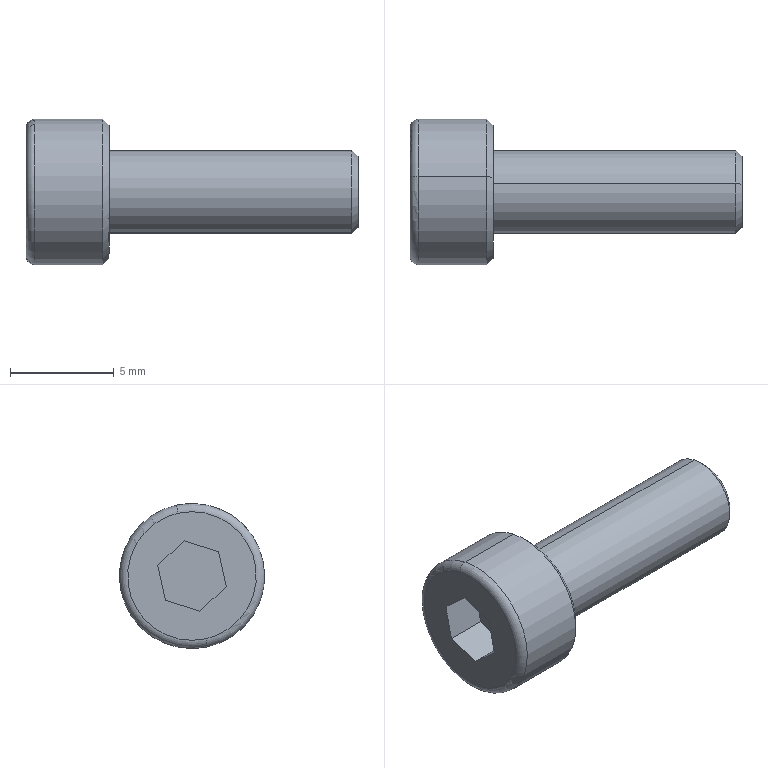Component | SolidWorks | SocketHeadCapScrew_M4_12-1 | 1 solid | 20 faces | box 16 x 7 x 7 mm | volume 287 mm3 | plane 10 | cone 4 | cylinder 4 | torus 2 | commonest cylinder face diameters 7 x2 4 x2
STEP:
#1=COLOUR_RGB('',0.7922,0.8196,0.9333);
#2=FILL_AREA_STYLE_COLOUR('',#1);
#3=FILL_AREA_STYLE('',(#2));
#4=SURFACE_STYLE_FILL_AREA(#3);
#5=SURFACE_SIDE_STYLE('',(#4));
#6=SURFACE_STYLE_USAGE(.BOTH.,#5);
#7=PRESENTATION_STYLE_ASSIGNMENT((#6));
#8=CARTESIAN_POINT('',(-0.1102,-0.2042,-1.204));
#9=VERTEX_POINT('',#8);
#10=CARTESIAN_POINT('',(-0.1102,-0.1502,-0.9575));
#11=VERTEX_POINT('',#10);
#12=CARTESIAN_POINT('',(-0.1102,-0.1772,-1.081));
#13=DIRECTION('',(1.,-0.,-0.));
#14=DIRECTION('',(0.,0.2142,0.9768));
#15=AXIS2_PLACEMENT_3D('',#12,#13,#14);
#16=CIRCLE('',#15,0.126);
#17=EDGE_CURVE('',#9,#11,#16,.T.);
#18=ORIENTED_EDGE('',*,*,#17,.F.);
#19=CARTESIAN_POINT('',(-0.122,-0.2067,-1.215));
#20=VERTEX_POINT('',#19);
#21=CARTESIAN_POINT('',(-0.122,-0.2067,-1.215));
#22=DIRECTION('',(-0.7071,-0.1515,-0.6907));
#23=VECTOR('',#22,39.37);
#24=LINE('',#21,#23);
#25=EDGE_CURVE('',#9,#20,#24,.T.);
#26=ORIENTED_EDGE('',*,*,#25,.T.);
#27=CARTESIAN_POINT('',(-0.122,-0.1476,-0.946));
#28=VERTEX_POINT('',#27);
#29=CARTESIAN_POINT('',(-0.122,-0.1772,-1.081));
#30=DIRECTION('',(-1.,0.,0.));
#31=DIRECTION('',(0.,0.2142,0.9768));
#32=AXIS2_PLACEMENT_3D('',#29,#30,#31);
#33=CIRCLE('',#32,0.1378);
#34=EDGE_CURVE('',#28,#20,#33,.T.);
#35=ORIENTED_EDGE('',*,*,#34,.F.);
#36=CARTESIAN_POINT('',(-0.122,-0.1476,-0.946));
#37=DIRECTION('',(-0.7071,0.1515,0.6907));
#38=VECTOR('',#37,39.37);
#39=LINE('',#36,#38);
#40=EDGE_CURVE('',#11,#28,#39,.T.);
#41=ORIENTED_EDGE('',*,*,#40,.F.);
#42=EDGE_LOOP('',(#18,#26,#35,#41));
#43=FACE_OUTER_BOUND('',#42,.T.);
#44=CARTESIAN_POINT('',(-0.122,-0.1772,-1.081));
#45=DIRECTION('',(-1.,0.,0.));
#46=DIRECTION('',(0.,0.2142,0.9768));
#47=AXIS2_PLACEMENT_3D('',#44,#45,#46);
#48=CONICAL_SURFACE('',#47,0.1378,0.7854);
#49=ADVANCED_FACE('',(#43),#48,.T.);
#50=CARTESIAN_POINT('',(0.3622,-0.1915,-1.146));
#51=VERTEX_POINT('',#50);
#52=CARTESIAN_POINT('',(0.3622,-0.1628,-1.015));
#53=VERTEX_POINT('',#52);
#54=CARTESIAN_POINT('',(0.3622,-0.1772,-1.081));
#55=DIRECTION('',(1.,-0.,-0.));
#56=DIRECTION('',(0.,0.2142,0.9768));
#57=AXIS2_PLACEMENT_3D('',#54,#55,#56);
#58=CIRCLE('',#57,0.06693);
#59=EDGE_CURVE('',#51,#53,#58,.T.);
#60=ORIENTED_EDGE('',*,*,#59,.F.);
#61=CARTESIAN_POINT('',(0.3504,-0.194,-1.157));
#62=VERTEX_POINT('',#61);
#63=CARTESIAN_POINT('',(0.3504,-0.194,-1.157));
#64=DIRECTION('',(-0.7071,-0.1515,-0.6907));
#65=VECTOR('',#64,39.37);
#66=LINE('',#63,#65);
#67=EDGE_CURVE('',#51,#62,#66,.T.);
#68=ORIENTED_EDGE('',*,*,#67,.T.);
#69=CARTESIAN_POINT('',(0.3504,-0.1603,-1.004));
#70=VERTEX_POINT('',#69);
#71=CARTESIAN_POINT('',(0.3504,-0.1772,-1.081));
#72=DIRECTION('',(-1.,0.,0.));
#73=DIRECTION('',(0.,0.2142,0.9768));
#74=AXIS2_PLACEMENT_3D('',#71,#72,#73);
#75=CIRCLE('',#74,0.07874);
#76=EDGE_CURVE('',#70,#62,#75,.T.);
#77=ORIENTED_EDGE('',*,*,#76,.F.);
#78=CARTESIAN_POINT('',(0.3504,-0.1603,-1.004));
#79=DIRECTION('',(-0.7071,0.1515,0.6907));
#80=VECTOR('',#79,39.37);
#81=LINE('',#78,#80);
#82=EDGE_CURVE('',#53,#70,#81,.T.);
#83=ORIENTED_EDGE('',*,*,#82,.F.);
#84=EDGE_LOOP('',(#60,#68,#77,#83));
#85=FACE_OUTER_BOUND('',#84,.T.);
#86=CARTESIAN_POINT('',(0.3504,-0.1772,-1.081));
#87=DIRECTION('',(-1.,0.,0.));
#88=DIRECTION('',(0.,0.2142,0.9768));
#89=AXIS2_PLACEMENT_3D('',#86,#87,#88);
#90=CONICAL_SURFACE('',#89,0.07874,0.7854);
#91=ADVANCED_FACE('',(#85),#90,.T.);
#92=CARTESIAN_POINT('',(-0.252,-0.1476,-0.946));
#93=VERTEX_POINT('',#92);
#94=CARTESIAN_POINT('',(-0.252,-0.2067,-1.215));
#95=VERTEX_POINT('',#94);
#96=CARTESIAN_POINT('',(-0.252,-0.1772,-1.081));
#97=DIRECTION('',(-1.,0.,0.));
#98=DIRECTION('',(0.,0.2142,0.9768));
#99=AXIS2_PLACEMENT_3D('',#96,#97,#98);
#100=CIRCLE('',#99,0.1378);
#101=EDGE_CURVE('',#93,#95,#100,.T.);
#102=ORIENTED_EDGE('',*,*,#101,.T.);
#103=CARTESIAN_POINT('',(-0.2677,-0.2033,-1.2));
#104=VERTEX_POINT('',#103);
#105=CARTESIAN_POINT('',(-0.252,-0.2033,-1.2));
#106=DIRECTION('',(0.,0.9768,-0.2142));
#107=DIRECTION('',(0.,0.2142,0.9768));
#108=AXIS2_PLACEMENT_3D('',#105,#106,#107);
#109=CIRCLE('',#108,0.01575);
#110=EDGE_CURVE('',#95,#104,#109,.T.);
#111=ORIENTED_EDGE('',*,*,#110,.T.);
#112=CARTESIAN_POINT('',(-0.2677,-0.151,-0.9613));
#113=VERTEX_POINT('',#112);
#114=CARTESIAN_POINT('',(-0.2677,-0.1772,-1.081));
#115=DIRECTION('',(-1.,0.,0.));
#116=DIRECTION('',(0.,0.2142,0.9768));
#117=AXIS2_PLACEMENT_3D('',#114,#115,#116);
#118=CIRCLE('',#117,0.122);
#119=EDGE_CURVE('',#113,#104,#118,.T.);
#120=ORIENTED_EDGE('',*,*,#119,.F.);
#121=CARTESIAN_POINT('',(-0.252,-0.151,-0.9613));
#122=DIRECTION('',(-0.,-0.9768,0.2142));
#123=DIRECTION('',(0.,-0.2142,-0.9768));
#124=AXIS2_PLACEMENT_3D('',#121,#122,#123);
#125=CIRCLE('',#124,0.01575);
#126=EDGE_CURVE('',#93,#113,#125,.T.);
#127=ORIENTED_EDGE('',*,*,#126,.F.);
#128=EDGE_LOOP('',(#102,#111,#120,#127));
#129=FACE_OUTER_BOUND('',#128,.T.);
#130=CARTESIAN_POINT('',(-0.252,-0.1772,-1.081));
#131=DIRECTION('',(-1.,0.,0.));
#132=DIRECTION('',(0.,0.2142,0.9768));
#133=AXIS2_PLACEMENT_3D('',#130,#131,#132);
#134=TOROIDAL_SURFACE('',#133,0.122,0.01575);
#135=ADVANCED_FACE('',(#129),#134,.T.);
#136=ORIENTED_EDGE('',*,*,#34,.T.);
#137=CARTESIAN_POINT('',(-0.2813,-0.2067,-1.215));
#138=DIRECTION('',(-1.,0.,0.));
#139=VECTOR('',#138,39.37);
#140=LINE('',#137,#139);
#141=EDGE_CURVE('',#20,#95,#140,.T.);
#142=ORIENTED_EDGE('',*,*,#141,.T.);
#143=ORIENTED_EDGE('',*,*,#101,.F.);
#144=CARTESIAN_POINT('',(-0.2813,-0.1476,-0.946));
#145=DIRECTION('',(-1.,0.,0.));
#146=VECTOR('',#145,39.37);
#147=LINE('',#144,#146);
#148=EDGE_CURVE('',#28,#93,#147,.T.);
#149=ORIENTED_EDGE('',*,*,#148,.F.);
#150=EDGE_LOOP('',(#136,#142,#143,#149));
#151=FACE_OUTER_BOUND('',#150,.T.);
#152=CARTESIAN_POINT('',(-0.2813,-0.1772,-1.081));
#153=DIRECTION('',(-1.,0.,0.));
#154=DIRECTION('',(0.,0.2142,0.9768));
#155=AXIS2_PLACEMENT_3D('',#152,#153,#154);
#156=CYLINDRICAL_SURFACE('',#155,0.1378);
#157=ADVANCED_FACE('',(#151),#156,.T.);
#158=ORIENTED_EDGE('',*,*,#76,.T.);
#159=CARTESIAN_POINT('',(-0.1102,-0.194,-1.157));
#160=VERTEX_POINT('',#159);
#161=CARTESIAN_POINT('',(-0.2813,-0.194,-1.157));
#162=DIRECTION('',(-1.,0.,0.));
#163=VECTOR('',#162,39.37);
#164=LINE('',#161,#163);
#165=EDGE_CURVE('',#62,#160,#164,.T.);
#166=ORIENTED_EDGE('',*,*,#165,.T.);
#167=CARTESIAN_POINT('',(-0.1102,-0.1603,-1.004));
#168=VERTEX_POINT('',#167);
#169=CARTESIAN_POINT('',(-0.1102,-0.1772,-1.081));
#170=DIRECTION('',(-1.,0.,0.));
#171=DIRECTION('',(0.,0.2142,0.9768));
#172=AXIS2_PLACEMENT_3D('',#169,#170,#171);
#173=CIRCLE('',#172,0.07874);
#174=EDGE_CURVE('',#168,#160,#173,.T.);
#175=ORIENTED_EDGE('',*,*,#174,.F.);
#176=CARTESIAN_POINT('',(-0.2813,-0.1603,-1.004));
#177=DIRECTION('',(-1.,0.,0.));
#178=VECTOR('',#177,39.37);
#179=LINE('',#176,#178);
#180=EDGE_CURVE('',#70,#168,#179,.T.);
#181=ORIENTED_EDGE('',*,*,#180,.F.);
#182=EDGE_LOOP('',(#158,#166,#175,#181));
#183=FACE_OUTER_BOUND('',#182,.T.);
#184=CARTESIAN_POINT('',(-0.2813,-0.1772,-1.081));
#185=DIRECTION('',(-1.,0.,0.));
#186=DIRECTION('',(0.,0.2142,0.9768));
#187=AXIS2_PLACEMENT_3D('',#184,#185,#186);
#188=CYLINDRICAL_SURFACE('',#187,0.07874);
#189=ADVANCED_FACE('',(#183),#188,.T.);
#190=CARTESIAN_POINT('',(0.3622,-0.1772,-1.081));
#191=DIRECTION('',(1.,-0.,-0.));
#192=DIRECTION('',(0.,0.2142,0.9768));
#193=AXIS2_PLACEMENT_3D('',#190,#191,#192);
#194=CIRCLE('',#193,0.06693);
#195=EDGE_CURVE('',#53,#51,#194,.T.);
#196=ORIENTED_EDGE('',*,*,#195,.T.);
#197=ORIENTED_EDGE('',*,*,#59,.T.);
#198=EDGE_LOOP('',(#196,#197));
#199=FACE_OUTER_BOUND('',#198,.T.);
#200=CARTESIAN_POINT('',(0.3622,-0.1003,-1.097));
#201=DIRECTION('',(-1.,0.,0.));
#202=DIRECTION('',(0.,0.2142,0.9768));
#203=AXIS2_PLACEMENT_3D('',#200,#201,#202);
#204=PLANE('',#203);
#205=ADVANCED_FACE('',(#199),#204,.F.);
#206=ORIENTED_EDGE('',*,*,#165,.F.);
#207=CARTESIAN_POINT('',(0.3504,-0.1772,-1.081));
#208=DIRECTION('',(-1.,0.,0.));
#209=DIRECTION('',(0.,0.2142,0.9768));
#210=AXIS2_PLACEMENT_3D('',#207,#208,#209);
#211=CIRCLE('',#210,0.07874);
#212=EDGE_CURVE('',#62,#70,#211,.T.);
#213=ORIENTED_EDGE('',*,*,#212,.T.);
#214=ORIENTED_EDGE('',*,*,#180,.T.);
#215=CARTESIAN_POINT('',(-0.1102,-0.1772,-1.081));
#216=DIRECTION('',(-1.,0.,0.));
#217=DIRECTION('',(0.,0.2142,0.9768));
#218=AXIS2_PLACEMENT_3D('',#215,#216,#217);
#219=CIRCLE('',#218,0.07874);
#220=EDGE_CURVE('',#160,#168,#219,.T.);
#221=ORIENTED_EDGE('',*,*,#220,.F.);
#222=EDGE_LOOP('',(#206,#213,#214,#221));
#223=FACE_OUTER_BOUND('',#222,.T.);
#224=CARTESIAN_POINT('',(-0.2813,-0.1772,-1.081));
#225=DIRECTION('',(-1.,0.,0.));
#226=DIRECTION('',(0.,0.2142,0.9768));
#227=AXIS2_PLACEMENT_3D('',#224,#225,#226);
#228=CYLINDRICAL_SURFACE('',#227,0.07874);
#229=ADVANCED_FACE('',(#223),#228,.T.);
#230=CARTESIAN_POINT('',(-0.1102,-0.1772,-1.081));
#231=DIRECTION('',(1.,-0.,-0.));
#232=DIRECTION('',(0.,0.2142,0.9768));
#233=AXIS2_PLACEMENT_3D('',#230,#231,#232);
#234=CIRCLE('',#233,0.126);
#235=EDGE_CURVE('',#11,#9,#234,.T.);
#236=ORIENTED_EDGE('',*,*,#235,.T.);
#237=ORIENTED_EDGE('',*,*,#17,.T.);
#238=EDGE_LOOP('',(#236,#237));
#239=FACE_OUTER_BOUND('',#238,.T.);
#240=ORIENTED_EDGE('',*,*,#174,.T.);
#241=ORIENTED_EDGE('',*,*,#220,.T.);
#242=EDGE_LOOP('',(#240,#241));
#243=FACE_BOUND('',#242,.T.);
#244=CARTESIAN_POINT('',(-0.1102,-0.04257,-1.11));
#245=DIRECTION('',(-1.,0.,0.));
#246=DIRECTION('',(0.,0.2142,0.9768));
#247=AXIS2_PLACEMENT_3D('',#244,#245,#246);
#248=PLANE('',#247);
#249=ADVANCED_FACE('',(#239,#243),#248,.F.);
#250=ORIENTED_EDGE('',*,*,#141,.F.);
#251=CARTESIAN_POINT('',(-0.122,-0.1772,-1.081));
#252=DIRECTION('',(-1.,0.,0.));
#253=DIRECTION('',(0.,0.2142,0.9768));
#254=AXIS2_PLACEMENT_3D('',#251,#252,#253);
#255=CIRCLE('',#254,0.1378);
#256=EDGE_CURVE('',#20,#28,#255,.T.);
#257=ORIENTED_EDGE('',*,*,#256,.T.);
#258=ORIENTED_EDGE('',*,*,#148,.T.);
#259=CARTESIAN_POINT('',(-0.252,-0.1772,-1.081));
#260=DIRECTION('',(-1.,0.,0.));
#261=DIRECTION('',(0.,0.2142,0.9768));
#262=AXIS2_PLACEMENT_3D('',#259,#260,#261);
#263=CIRCLE('',#262,0.1378);
#264=EDGE_CURVE('',#95,#93,#263,.T.);
#265=ORIENTED_EDGE('',*,*,#264,.F.);
#266=EDGE_LOOP('',(#250,#257,#258,#265));
#267=FACE_OUTER_BOUND('',#266,.T.);
#268=CARTESIAN_POINT('',(-0.2813,-0.1772,-1.081));
#269=DIRECTION('',(-1.,0.,0.));
#270=DIRECTION('',(0.,0.2142,0.9768));
#271=AXIS2_PLACEMENT_3D('',#268,#269,#270);
#272=CYLINDRICAL_SURFACE('',#271,0.1378);
#273=ADVANCED_FACE('',(#267),#272,.T.);
#274=ORIENTED_EDGE('',*,*,#110,.F.);
#275=ORIENTED_EDGE('',*,*,#264,.T.);
#276=ORIENTED_EDGE('',*,*,#126,.T.);
#277=CARTESIAN_POINT('',(-0.2677,-0.1772,-1.081));
#278=DIRECTION('',(-1.,0.,0.));
#279=DIRECTION('',(0.,0.2142,0.9768));
#280=AXIS2_PLACEMENT_3D('',#277,#278,#279);
#281=CIRCLE('',#280,0.122);
#282=EDGE_CURVE('',#104,#113,#281,.T.);
#283=ORIENTED_EDGE('',*,*,#282,.F.);
#284=EDGE_LOOP('',(#274,#275,#276,#283));
#285=FACE_OUTER_BOUND('',#284,.T.);
#286=CARTESIAN_POINT('',(-0.252,-0.1772,-1.081));
#287=DIRECTION('',(-1.,0.,0.));
#288=DIRECTION('',(0.,0.2142,0.9768));
#289=AXIS2_PLACEMENT_3D('',#286,#287,#288);
#290=TOROIDAL_SURFACE('',#289,0.122,0.01575);
#291=ADVANCED_FACE('',(#285),#290,.T.);
#292=CARTESIAN_POINT('',(-0.2677,-0.1626,-1.014));
#293=VERTEX_POINT('',#292);
#294=CARTESIAN_POINT('',(-0.2677,-0.1122,-1.06));
#295=VERTEX_POINT('',#294);
#296=CARTESIAN_POINT('',(-0.2677,-0.1626,-1.014));
#297=DIRECTION('',(-0.,0.7388,-0.6739));
#298=VECTOR('',#297,39.37);
#299=LINE('',#296,#298);
#300=EDGE_CURVE('',#293,#295,#299,.T.);
#301=ORIENTED_EDGE('',*,*,#300,.F.);
#302=CARTESIAN_POINT('',(-0.2677,-0.2275,-1.035));
#303=VERTEX_POINT('',#302);
#304=CARTESIAN_POINT('',(-0.2677,-0.2275,-1.035));
#305=DIRECTION('',(0.,0.953,0.3029));
#306=VECTOR('',#305,39.37);
#307=LINE('',#304,#306);
#308=EDGE_CURVE('',#303,#293,#307,.T.);
#309=ORIENTED_EDGE('',*,*,#308,.F.);
#310=CARTESIAN_POINT('',(-0.2677,-0.2422,-1.101));
#311=VERTEX_POINT('',#310);
#312=CARTESIAN_POINT('',(-0.2677,-0.2422,-1.101));
#313=DIRECTION('',(0.,0.2142,0.9768));
#314=VECTOR('',#313,39.37);
#315=LINE('',#312,#314);
#316=EDGE_CURVE('',#311,#303,#315,.T.);
#317=ORIENTED_EDGE('',*,*,#316,.F.);
#318=CARTESIAN_POINT('',(-0.2677,-0.1918,-1.147));
#319=VERTEX_POINT('',#318);
#320=CARTESIAN_POINT('',(-0.2677,-0.1918,-1.147));
#321=DIRECTION('',(0.,-0.7388,0.6739));
#322=VECTOR('',#321,39.37);
#323=LINE('',#320,#322);
#324=EDGE_CURVE('',#319,#311,#323,.T.);
#325=ORIENTED_EDGE('',*,*,#324,.F.);
#326=CARTESIAN_POINT('',(-0.2677,-0.1268,-1.127));
#327=VERTEX_POINT('',#326);
#328=CARTESIAN_POINT('',(-0.2677,-0.1268,-1.127));
#329=DIRECTION('',(-0.,-0.953,-0.3029));
#330=VECTOR('',#329,39.37);
#331=LINE('',#328,#330);
#332=EDGE_CURVE('',#327,#319,#331,.T.);
#333=ORIENTED_EDGE('',*,*,#332,.F.);
#334=CARTESIAN_POINT('',(-0.2677,-0.1122,-1.06));
#335=DIRECTION('',(-0.,-0.2142,-0.9768));
#336=VECTOR('',#335,39.37);
#337=LINE('',#334,#336);
#338=EDGE_CURVE('',#295,#327,#337,.T.);
#339=ORIENTED_EDGE('',*,*,#338,.F.);
#340=EDGE_LOOP('',(#301,#309,#317,#325,#333,#339));
#341=FACE_BOUND('',#340,.T.);
#342=ORIENTED_EDGE('',*,*,#119,.T.);
#343=ORIENTED_EDGE('',*,*,#282,.T.);
#344=EDGE_LOOP('',(#342,#343));
#345=FACE_OUTER_BOUND('',#344,.T.);
#346=CARTESIAN_POINT('',(-0.2677,-0.1772,-1.081));
#347=DIRECTION('',(1.,-0.,-0.));
#348=DIRECTION('',(-0.,-0.2142,-0.9768));
#349=AXIS2_PLACEMENT_3D('',#346,#347,#348);
#350=PLANE('',#349);
#351=ADVANCED_FACE('',(#341,#345),#350,.F.);
#352=ORIENTED_EDGE('',*,*,#308,.T.);
#353=CARTESIAN_POINT('',(-0.189,-0.1626,-1.014));
#354=VERTEX_POINT('',#353);
#355=CARTESIAN_POINT('',(-0.189,-0.1626,-1.014));
#356=DIRECTION('',(-1.,0.,0.));
#357=VECTOR('',#356,39.37);
#358=LINE('',#355,#357);
#359=EDGE_CURVE('',#354,#293,#358,.T.);
#360=ORIENTED_EDGE('',*,*,#359,.F.);
#361=CARTESIAN_POINT('',(-0.189,-0.2275,-1.035));
#362=VERTEX_POINT('',#361);
#363=CARTESIAN_POINT('',(-0.189,-0.2275,-1.035));
#364=DIRECTION('',(0.,0.953,0.3029));
#365=VECTOR('',#364,39.37);
#366=LINE('',#363,#365);
#367=EDGE_CURVE('',#362,#354,#366,.T.);
#368=ORIENTED_EDGE('',*,*,#367,.F.);
#369=CARTESIAN_POINT('',(-0.189,-0.2275,-1.035));
#370=DIRECTION('',(-1.,0.,0.));
#371=VECTOR('',#370,39.37);
#372=LINE('',#369,#371);
#373=EDGE_CURVE('',#362,#303,#372,.T.);
#374=ORIENTED_EDGE('',*,*,#373,.T.);
#375=EDGE_LOOP('',(#352,#360,#368,#374));
#376=FACE_OUTER_BOUND('',#375,.T.);
#377=CARTESIAN_POINT('',(-0.189,-0.2275,-1.035));
#378=DIRECTION('',(0.,-0.3029,0.953));
#379=DIRECTION('',(-0.,-0.953,-0.3029));
#380=AXIS2_PLACEMENT_3D('',#377,#378,#379);
#381=PLANE('',#380);
#382=ADVANCED_FACE('',(#376),#381,.F.);
#383=ORIENTED_EDGE('',*,*,#316,.T.);
#384=ORIENTED_EDGE('',*,*,#373,.F.);
#385=CARTESIAN_POINT('',(-0.189,-0.2422,-1.101));
#386=VERTEX_POINT('',#385);
#387=CARTESIAN_POINT('',(-0.189,-0.2422,-1.101));
#388=DIRECTION('',(0.,0.2142,0.9768));
#389=VECTOR('',#388,39.37);
#390=LINE('',#387,#389);
#391=EDGE_CURVE('',#386,#362,#390,.T.);
#392=ORIENTED_EDGE('',*,*,#391,.F.);
#393=CARTESIAN_POINT('',(-0.189,-0.2422,-1.101));
#394=DIRECTION('',(-1.,0.,0.));
#395=VECTOR('',#394,39.37);
#396=LINE('',#393,#395);
#397=EDGE_CURVE('',#386,#311,#396,.T.);
#398=ORIENTED_EDGE('',*,*,#397,.T.);
#399=EDGE_LOOP('',(#383,#384,#392,#398));
#400=FACE_OUTER_BOUND('',#399,.T.);
#401=CARTESIAN_POINT('',(-0.189,-0.2422,-1.101));
#402=DIRECTION('',(-0.,-0.9768,0.2142));
#403=DIRECTION('',(-0.,-0.2142,-0.9768));
#404=AXIS2_PLACEMENT_3D('',#401,#402,#403);
#405=PLANE('',#404);
#406=ADVANCED_FACE('',(#400),#405,.F.);
#407=ORIENTED_EDGE('',*,*,#324,.T.);
#408=ORIENTED_EDGE('',*,*,#397,.F.);
#409=CARTESIAN_POINT('',(-0.189,-0.1918,-1.147));
#410=VERTEX_POINT('',#409);
#411=CARTESIAN_POINT('',(-0.189,-0.1918,-1.147));
#412=DIRECTION('',(0.,-0.7388,0.6739));
#413=VECTOR('',#412,39.37);
#414=LINE('',#411,#413);
#415=EDGE_CURVE('',#410,#386,#414,.T.);
#416=ORIENTED_EDGE('',*,*,#415,.F.);
#417=CARTESIAN_POINT('',(-0.189,-0.1918,-1.147));
#418=DIRECTION('',(-1.,0.,0.));
#419=VECTOR('',#418,39.37);
#420=LINE('',#417,#419);
#421=EDGE_CURVE('',#410,#319,#420,.T.);
#422=ORIENTED_EDGE('',*,*,#421,.T.);
#423=EDGE_LOOP('',(#407,#408,#416,#422));
#424=FACE_OUTER_BOUND('',#423,.T.);
#425=CARTESIAN_POINT('',(-0.189,-0.1918,-1.147));
#426=DIRECTION('',(-0.,-0.6739,-0.7388));
#427=DIRECTION('',(-0.,0.7388,-0.6739));
#428=AXIS2_PLACEMENT_3D('',#425,#426,#427);
#429=PLANE('',#428);
#430=ADVANCED_FACE('',(#424),#429,.F.);
#431=ORIENTED_EDGE('',*,*,#332,.T.);
#432=ORIENTED_EDGE('',*,*,#421,.F.);
#433=CARTESIAN_POINT('',(-0.189,-0.1268,-1.127));
#434=VERTEX_POINT('',#433);
#435=CARTESIAN_POINT('',(-0.189,-0.1268,-1.127));
#436=DIRECTION('',(-0.,-0.953,-0.3029));
#437=VECTOR('',#436,39.37);
#438=LINE('',#435,#437);
#439=EDGE_CURVE('',#434,#410,#438,.T.);
#440=ORIENTED_EDGE('',*,*,#439,.F.);
#441=CARTESIAN_POINT('',(-0.189,-0.1268,-1.127));
#442=DIRECTION('',(-1.,0.,0.));
#443=VECTOR('',#442,39.37);
#444=LINE('',#441,#443);
#445=EDGE_CURVE('',#434,#327,#444,.T.);
#446=ORIENTED_EDGE('',*,*,#445,.T.);
#447=EDGE_LOOP('',(#431,#432,#440,#446));
#448=FACE_OUTER_BOUND('',#447,.T.);
#449=CARTESIAN_POINT('',(-0.189,-0.1268,-1.127));
#450=DIRECTION('',(-0.,0.3029,-0.953));
#451=DIRECTION('',(0.,0.953,0.3029));
#452=AXIS2_PLACEMENT_3D('',#449,#450,#451);
#453=PLANE('',#452);
#454=ADVANCED_FACE('',(#448),#453,.F.);
#455=ORIENTED_EDGE('',*,*,#338,.T.);
#456=ORIENTED_EDGE('',*,*,#445,.F.);
#457=CARTESIAN_POINT('',(-0.189,-0.1122,-1.06));
#458=VERTEX_POINT('',#457);
#459=CARTESIAN_POINT('',(-0.189,-0.1122,-1.06));
#460=DIRECTION('',(-0.,-0.2142,-0.9768));
#461=VECTOR('',#460,39.37);
#462=LINE('',#459,#461);
#463=EDGE_CURVE('',#458,#434,#462,.T.);
#464=ORIENTED_EDGE('',*,*,#463,.F.);
#465=CARTESIAN_POINT('',(-0.189,-0.1122,-1.06));
#466=DIRECTION('',(-1.,0.,0.));
#467=VECTOR('',#466,39.37);
#468=LINE('',#465,#467);
#469=EDGE_CURVE('',#458,#295,#468,.T.);
#470=ORIENTED_EDGE('',*,*,#469,.T.);
#471=EDGE_LOOP('',(#455,#456,#464,#470));
#472=FACE_OUTER_BOUND('',#471,.T.);
#473=CARTESIAN_POINT('',(-0.189,-0.1122,-1.06));
#474=DIRECTION('',(0.,0.9768,-0.2142));
#475=DIRECTION('',(0.,0.2142,0.9768));
#476=AXIS2_PLACEMENT_3D('',#473,#474,#475);
#477=PLANE('',#476);
#478=ADVANCED_FACE('',(#472),#477,.F.);
#479=ORIENTED_EDGE('',*,*,#300,.T.);
#480=ORIENTED_EDGE('',*,*,#469,.F.);
#481=CARTESIAN_POINT('',(-0.189,-0.1626,-1.014));
#482=DIRECTION('',(-0.,0.7388,-0.6739));
#483=VECTOR('',#482,39.37);
#484=LINE('',#481,#483);
#485=EDGE_CURVE('',#354,#458,#484,.T.);
#486=ORIENTED_EDGE('',*,*,#485,.F.);
#487=ORIENTED_EDGE('',*,*,#359,.T.);
#488=EDGE_LOOP('',(#479,#480,#486,#487));
#489=FACE_OUTER_BOUND('',#488,.T.);
#490=CARTESIAN_POINT('',(-0.189,-0.1626,-1.014));
#491=DIRECTION('',(0.,0.6739,0.7388));
#492=DIRECTION('',(0.,-0.7388,0.6739));
#493=AXIS2_PLACEMENT_3D('',#490,#491,#492);
#494=PLANE('',#493);
#495=ADVANCED_FACE('',(#489),#494,.F.);
#496=ORIENTED_EDGE('',*,*,#367,.T.);
#497=ORIENTED_EDGE('',*,*,#485,.T.);
#498=ORIENTED_EDGE('',*,*,#463,.T.);
#499=ORIENTED_EDGE('',*,*,#439,.T.);
#500=ORIENTED_EDGE('',*,*,#415,.T.);
#501=ORIENTED_EDGE('',*,*,#391,.T.);
#502=EDGE_LOOP('',(#496,#497,#498,#499,#500,#501));
#503=FACE_OUTER_BOUND('',#502,.T.);
#504=CARTESIAN_POINT('',(-0.189,-0.2275,-1.035));
#505=DIRECTION('',(1.,-0.,-0.));
#506=DIRECTION('',(-0.,-0.2142,-0.9768));
#507=AXIS2_PLACEMENT_3D('',#504,#505,#506);
#508=PLANE('',#507);
#509=ADVANCED_FACE('',(#503),#508,.F.);
#510=ORIENTED_EDGE('',*,*,#67,.F.);
#511=ORIENTED_EDGE('',*,*,#195,.F.);
#512=ORIENTED_EDGE('',*,*,#82,.T.);
#513=ORIENTED_EDGE('',*,*,#212,.F.);
#514=EDGE_LOOP('',(#510,#511,#512,#513));
#515=FACE_OUTER_BOUND('',#514,.T.);
#516=CARTESIAN_POINT('',(0.3504,-0.1772,-1.081));
#517=DIRECTION('',(-1.,0.,0.));
#518=DIRECTION('',(0.,0.2142,0.9768));
#519=AXIS2_PLACEMENT_3D('',#516,#517,#518);
#520=CONICAL_SURFACE('',#519,0.07874,0.7854);
#521=ADVANCED_FACE('',(#515),#520,.T.);
#522=ORIENTED_EDGE('',*,*,#25,.F.);
#523=ORIENTED_EDGE('',*,*,#235,.F.);
#524=ORIENTED_EDGE('',*,*,#40,.T.);
#525=ORIENTED_EDGE('',*,*,#256,.F.);
#526=EDGE_LOOP('',(#522,#523,#524,#525));
#527=FACE_OUTER_BOUND('',#526,.T.);
#528=CARTESIAN_POINT('',(-0.122,-0.1772,-1.081));
#529=DIRECTION('',(-1.,0.,0.));
#530=DIRECTION('',(0.,0.2142,0.9768));
#531=AXIS2_PLACEMENT_3D('',#528,#529,#530);
#532=CONICAL_SURFACE('',#531,0.1378,0.7854);
#533=ADVANCED_FACE('',(#527),#532,.T.);
#534=CLOSED_SHELL('',(#49,#91,#135,#157,#189,#205,#229,#249,#273,#291,#351,#382,#406,#430,#454,#478,#495,#509,#521,#533));
#535=MANIFOLD_SOLID_BREP('',#534);
#536=STYLED_ITEM('',(#7),#535);
#537=PRESENTATION_LAYER_ASSIGNMENT('','',(#536));
#538=CARTESIAN_POINT('',(0.,0.,0.));
#539=DIRECTION('',(0.,0.,1.));
#540=DIRECTION('',(1.,0.,0.));
#541=AXIS2_PLACEMENT_3D('',#538,#539,#540);
#542=(LENGTH_UNIT()NAMED_UNIT(*)SI_UNIT($,.METRE.));
#543=LENGTH_MEASURE_WITH_UNIT(LENGTH_MEASURE(0.0254),#542);
#544=DIMENSIONAL_EXPONENTS(1.,0.,0.,0.,0.,0.,0.);
#545=(CONVERSION_BASED_UNIT('',#543)LENGTH_UNIT()NAMED_UNIT(#544));
#546=UNCERTAINTY_MEASURE_WITH_UNIT(LENGTH_MEASURE(0.00001),#545,'','');
#547=(NAMED_UNIT(*)PLANE_ANGLE_UNIT()SI_UNIT($,.RADIAN.));
#548=(NAMED_UNIT(*)SI_UNIT($,.STERADIAN.)SOLID_ANGLE_UNIT());
#549=(GEOMETRIC_REPRESENTATION_CONTEXT(3)GLOBAL_UNCERTAINTY_ASSIGNED_CONTEXT((#546))GLOBAL_UNIT_ASSIGNED_CONTEXT((#545,#547,#548))REPRESENTATION_CONTEXT('',''));
#550=ADVANCED_BREP_SHAPE_REPRESENTATION('',(#535,#541),#549);
#551=(LENGTH_UNIT()NAMED_UNIT(*)SI_UNIT($,.METRE.));
#552=LENGTH_MEASURE_WITH_UNIT(LENGTH_MEASURE(0.0254),#551);
#553=DIMENSIONAL_EXPONENTS(1.,0.,0.,0.,0.,0.,0.);
#554=(CONVERSION_BASED_UNIT('',#552)LENGTH_UNIT()NAMED_UNIT(#553));
#555=UNCERTAINTY_MEASURE_WITH_UNIT(LENGTH_MEASURE(0.00001),#554,'','');
#556=(NAMED_UNIT(*)PLANE_ANGLE_UNIT()SI_UNIT($,.RADIAN.));
#557=(NAMED_UNIT(*)SI_UNIT($,.STERADIAN.)SOLID_ANGLE_UNIT());
#558=(GEOMETRIC_REPRESENTATION_CONTEXT(3)GLOBAL_UNCERTAINTY_ASSIGNED_CONTEXT((#555))GLOBAL_UNIT_ASSIGNED_CONTEXT((#554,#556,#557))REPRESENTATION_CONTEXT('',''));
#559=MECHANICAL_DESIGN_GEOMETRIC_PRESENTATION_REPRESENTATION('',(#536),#558);